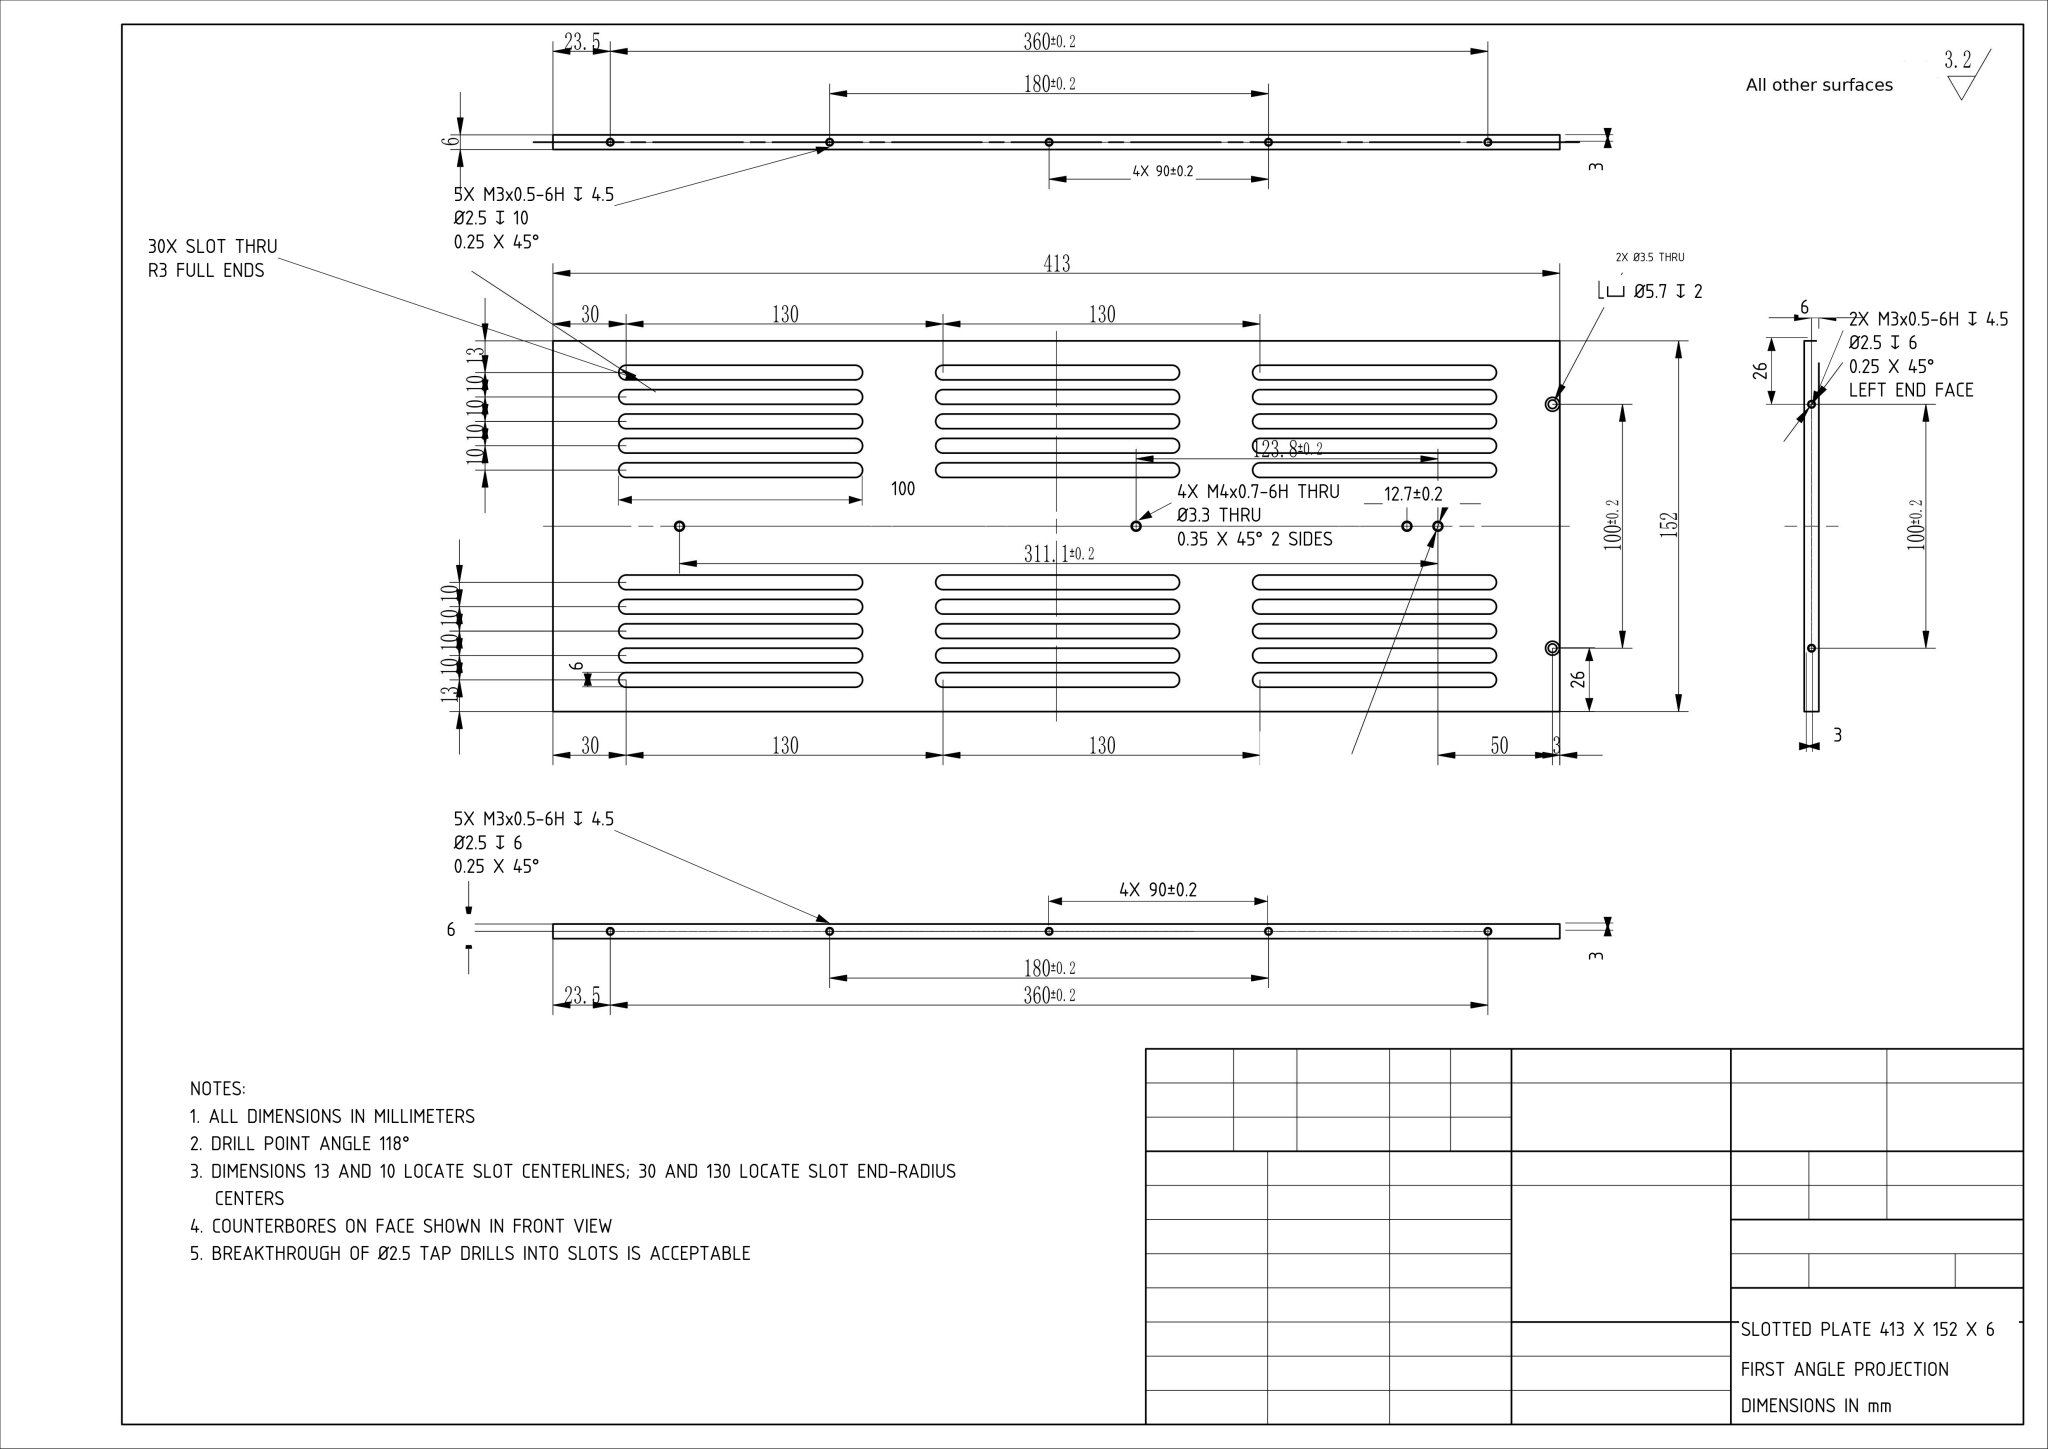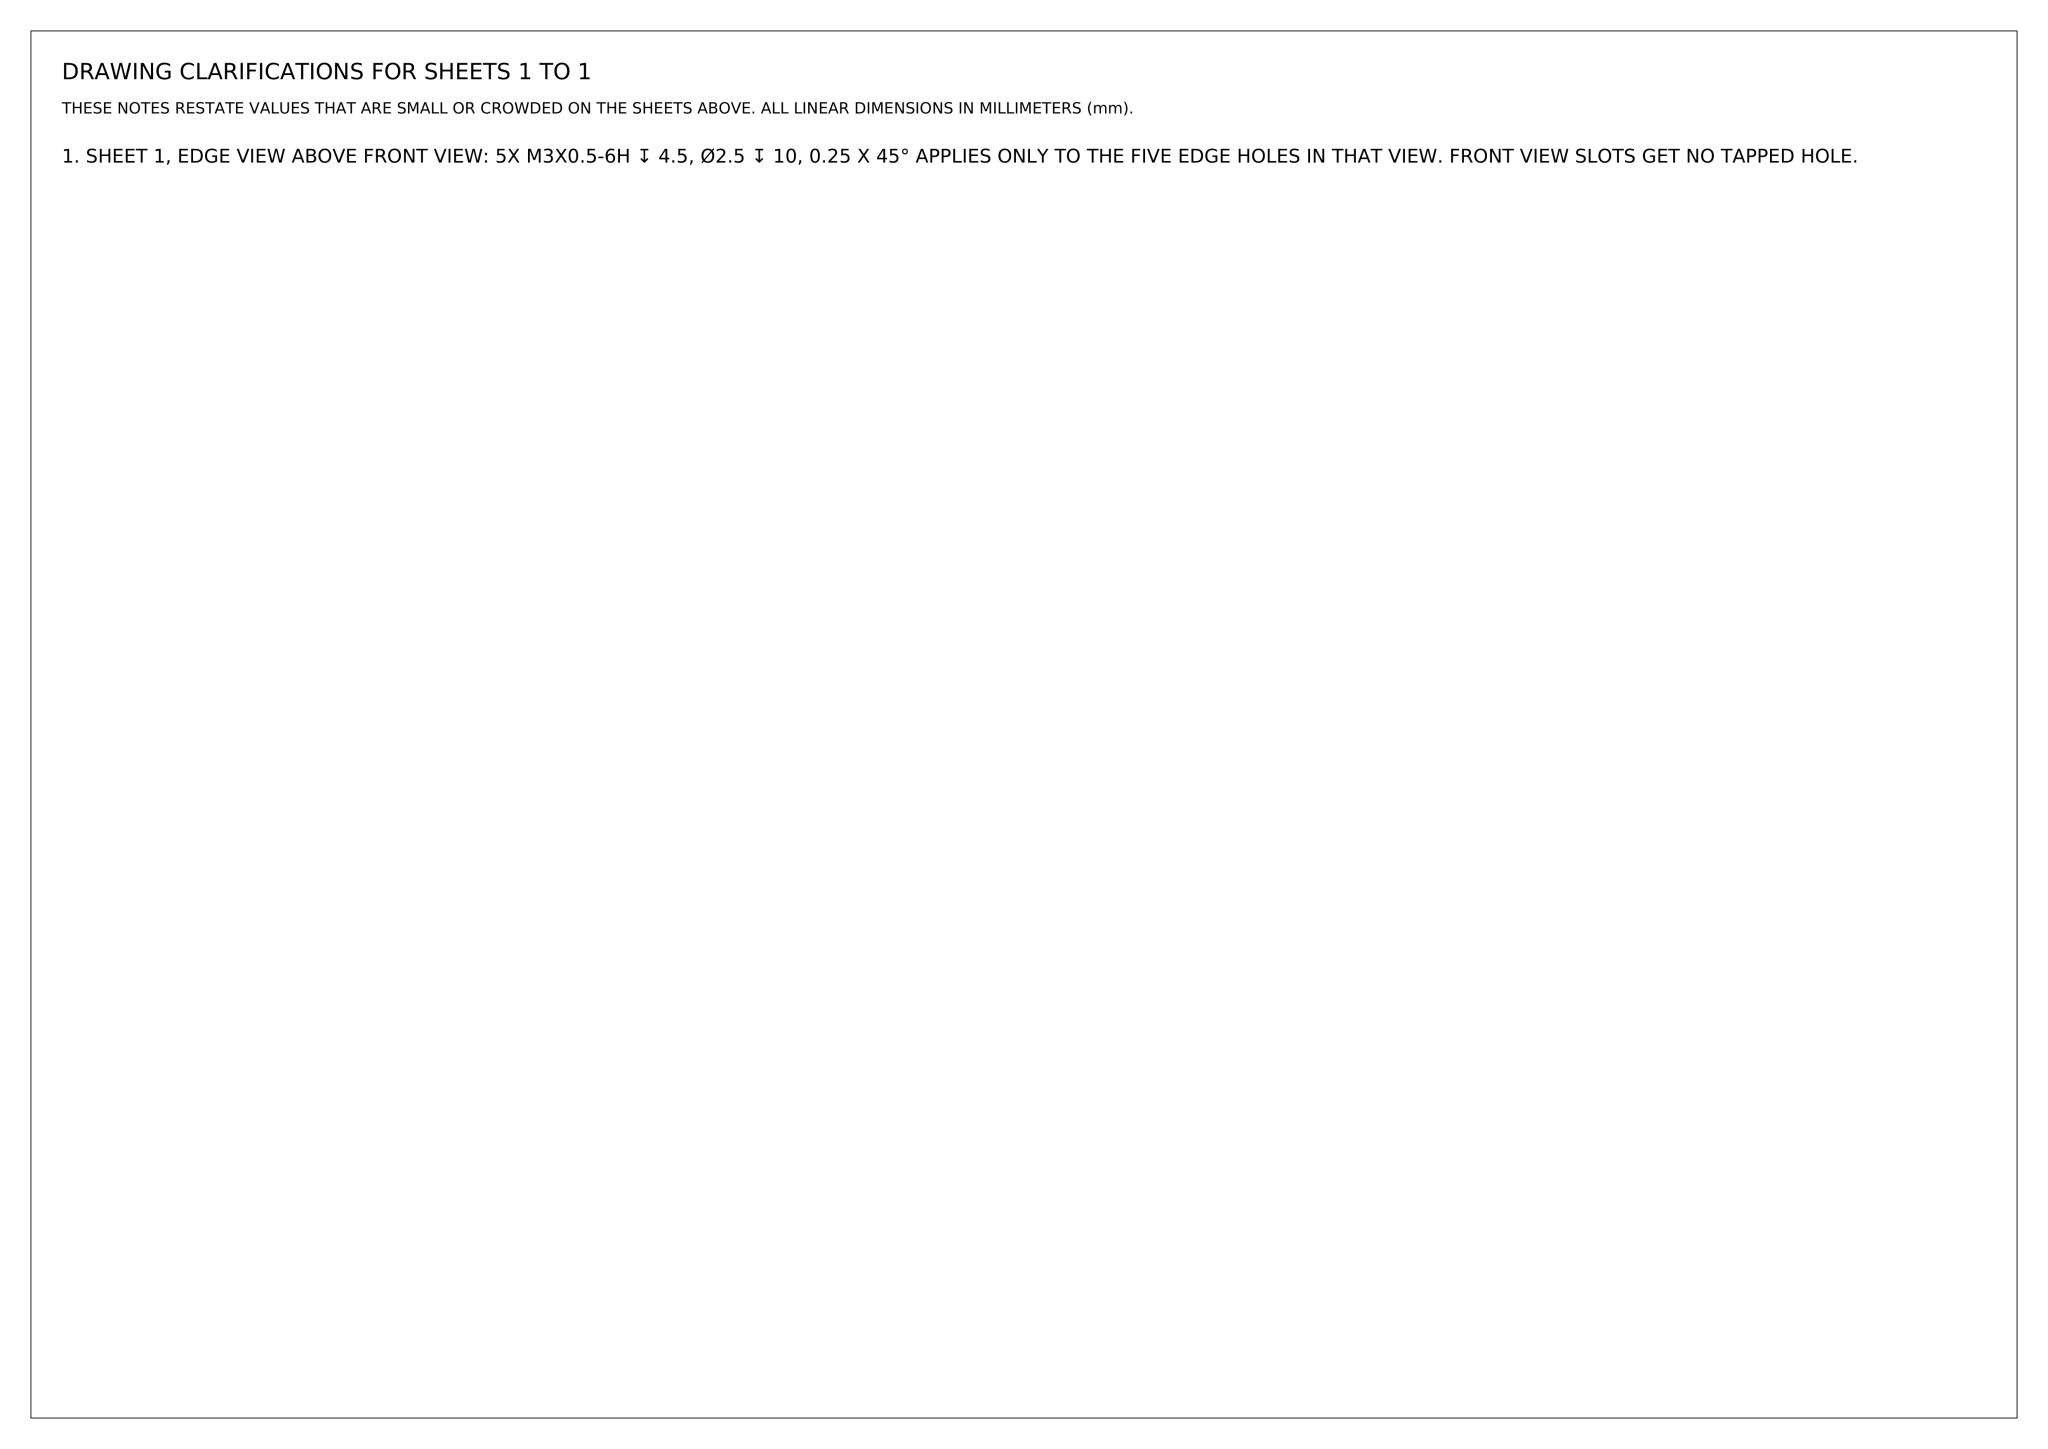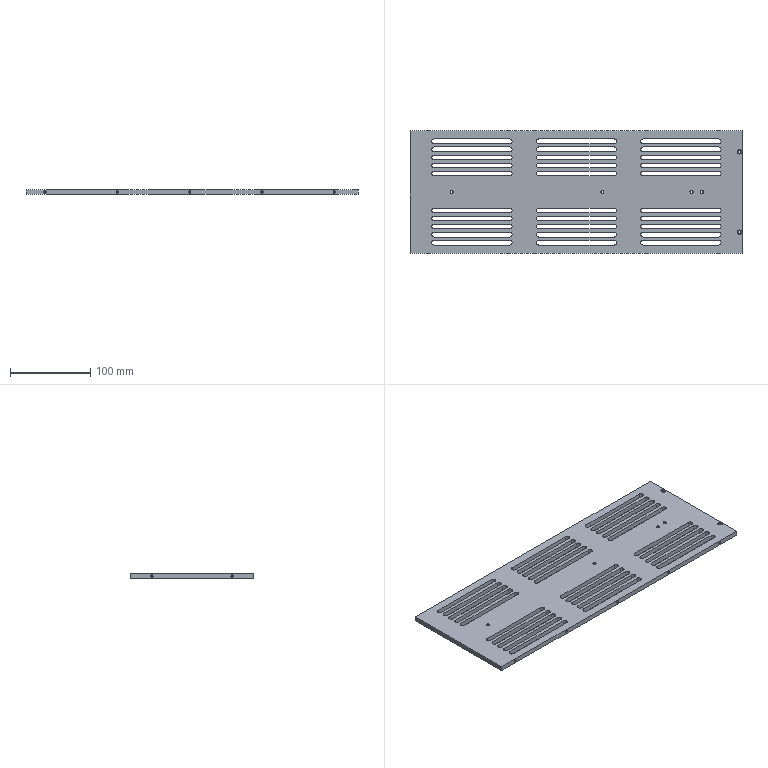Part | NX | mm | 1 solid | 178 faces | box 413 x 152 x 6 mm | volume 269191 mm3 | cylinder 80 | plane 69 | cone 28 | spline 1 | commonest cylinder face diameters 6 x60 2.5 x12 3.3 x4 3.5 x2 5.7 x2